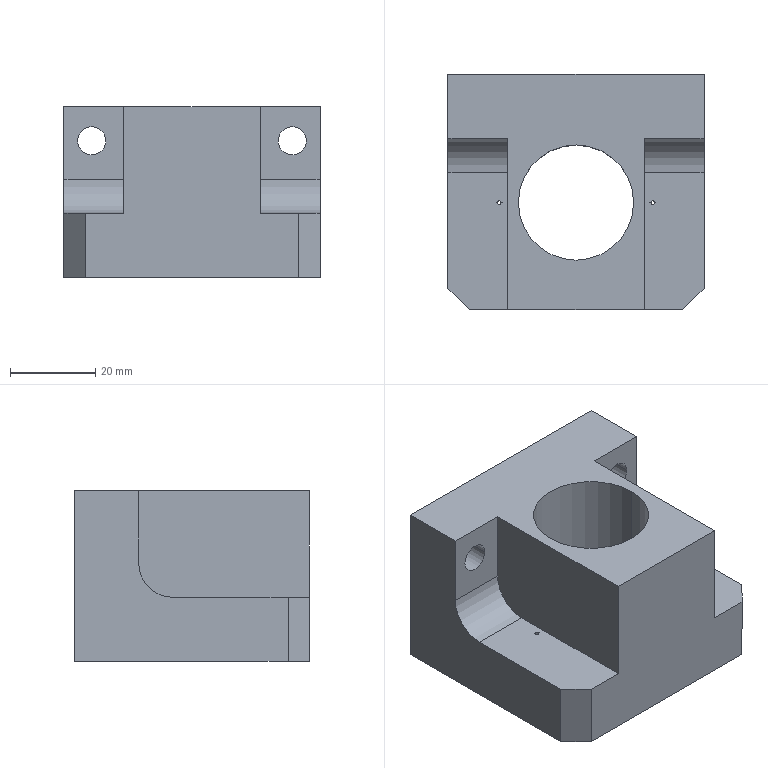Component | SolidWorks | OPW-05-010-1 | 1 solid | 38 faces | box 60 x 55 x 40 mm | volume 79282 mm3 | cylinder 16 | plane 14 | cone 8 | commonest cylinder face diameters 4.2 x8 6.6 x4 27 x2 16 x2
build123d program:
from build123d import *

# Parameters (mm, degrees)
SKETCH1_W                  = 60
SKETCH1_H                  = 55
BOSS_EXTRUDE1_DEPTH        = 20
CUT_EXTRUDE1_REACH         = 59.064
SKETCH2_R                  = 13.5
CIRPATTERN1_COUNT          = 4
SKETCH5_W                  = 25
SKETCH5_H                  = 40
CUT_EXTRUDE2_DEPTH         = 14
FILLET1_R                  = 8
FILLET1_OF_MIRROR1_R       = 8
F_6_6_6_6_DIAMETER_HOLE1_D = 6.6
CHAMFER2_SIZE              = 5


with BuildPart() as part:
    # Sketch1 → Boss-Extrude1 (new, symmetric)
    with BuildSketch(Plane(origin=(0, 0, 0), x_dir=(0, 0, -1), z_dir=(1, 0, 0))):
        Rectangle(SKETCH1_W, SKETCH1_H)
    extrude(amount=BOSS_EXTRUDE1_DEPTH, both=True)

    # Sketch2 → Cut-Extrude1 (cut, up to next)
    with BuildSketch(Plane(origin=(20, 0, 0), x_dir=(0, 0, -1), z_dir=(1, 0, 0)), mode=Mode.PRIVATE) as cut_extrude1_sk1:
        with Locations((0, -2.5)):
            Circle(SKETCH2_R)
    cut_extrude1_tool1 = extrude(cut_extrude1_sk1.sketch, amount=-CUT_EXTRUDE1_REACH, mode=Mode.PRIVATE) & part.part
    add(cut_extrude1_tool1.solids().sort_by_distance((20, -2.5, 0))[0], mode=Mode.SUBTRACT)

    # Sketch3 → M5 Tapped Hole1 (revolve, cut)
    with BuildSketch(Plane(origin=(20, 15.5, 0), x_dir=(0, 0, -1), z_dir=(0, 1, 0))):
        Polygon((0, 0), (0, 15.262), (2.1, 14), (2.1, 0), align=None)
    m5_tapped_hole1 = revolve(axis=Axis((26.35, 15.5, 0), (-1, 0, 0)), mode=Mode.SUBTRACT)

    # CirPattern1: M5 Tapped Hole1 ×4 about axis
    cirpattern1_axis = Axis((0, -2.5, 0), (1, 0, 0))
    for i in range(1, CIRPATTERN1_COUNT):
        add(m5_tapped_hole1.rotate(cirpattern1_axis, i * 360 / CIRPATTERN1_COUNT), mode=Mode.SUBTRACT)

    # Sketch5 → Cut-Extrude2 (cut)
    with BuildSketch(Plane.XY.offset(30)):
        with Locations((-7.5, -7.5)):
            Rectangle(SKETCH5_W, SKETCH5_H)
    cut_extrude2 = extrude(amount=-CUT_EXTRUDE2_DEPTH, mode=Mode.SUBTRACT)

    # Fillet1
    fillet1_edges = [part.edges().sort_by_distance(p)[0] for p in [
        (5, 12.5, 23),
    ]]
    fillet(fillet1_edges, radius=FILLET1_R)

    # Mirror1: Cut-Extrude2 across plane
    add(cut_extrude2.mirror(Plane.XY), mode=Mode.SUBTRACT)

    # Fillet1 of Mirror1
    fillet1_of_mirror1_edges = [part.edges().sort_by_distance(p)[0] for p in [
        (5, 12.5, -23),
    ]]
    fillet(fillet1_of_mirror1_edges, radius=FILLET1_OF_MIRROR1_R)

    # 6.6 _6.6_ Diameter Hole1 (through all)
    with Locations(Plane.XZ.offset(-12.5)):
        with Locations((-12, 23.5), (-12, -23.5)):
            Hole(F_6_6_6_6_DIAMETER_HOLE1_D / 2)

    # Chamfer2
    chamfer2_edges = [part.edges().sort_by_distance(p)[0] for p in [
        (12.5, -27.5, -30),
        (12.5, -27.5, 30),
    ]]
    chamfer(chamfer2_edges, length=CHAMFER2_SIZE)


solid = part.part

# Placed as in the assembly
solid = solid.moved(Location((0.5965, 14.499, -10), (0, 90, 0)))